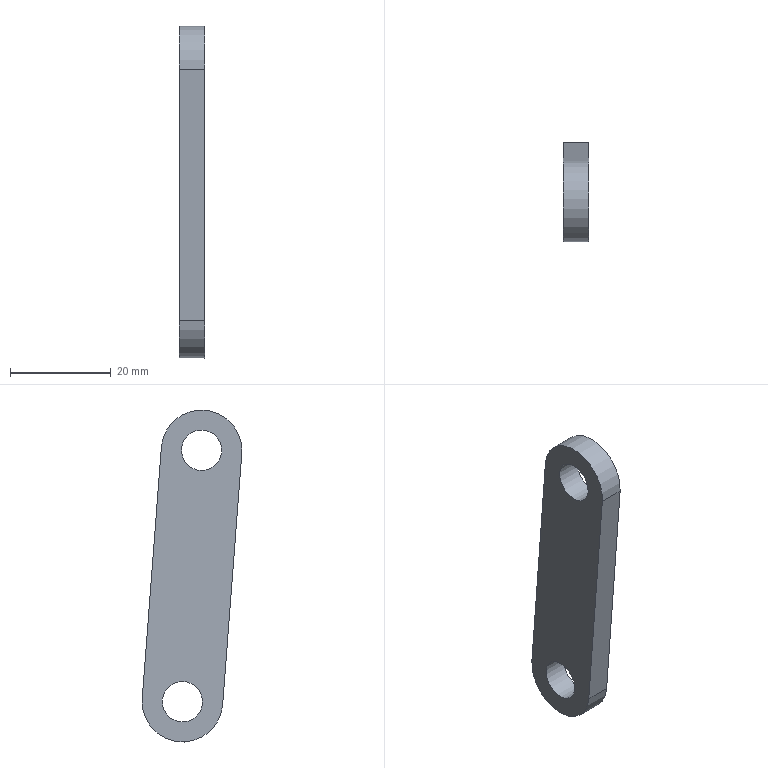Component | NX | JAWLINK2_3 | 1 solid | 8 faces | box 5 x 19.79 x 65.86 mm | volume 4503 mm3 | plane 4 | cylinder 4 | commonest cylinder face diameters 16 x2 8 x2
STEP:
#1=CARTESIAN_POINT('',(0.,0.,0.));
#2=DIRECTION('',(0.,0.,1.));
#3=DIRECTION('',(1.,0.,0.));
#4=AXIS2_PLACEMENT_3D('',#1,#2,#3);
#5=CARTESIAN_POINT('',(-17.89,-45.538,-245.161));
#6=VERTEX_POINT('',#5);
#7=CARTESIAN_POINT('',(-17.89,-41.549,-244.858));
#8=DIRECTION('',(-1.,0.,0.));
#9=DIRECTION('',(0.,-0.9971,-0.07581));
#10=AXIS2_PLACEMENT_3D('',#7,#8,#9);
#11=CIRCLE('',#10,4.);
#12=CARTESIAN_POINT('',(-17.89,-39.654,-269.786));
#13=DIRECTION('',(1.,0.,0.));
#14=DIRECTION('',(0.,0.9971,0.07581));
#15=AXIS2_PLACEMENT_3D('',#12,#13,#14);
#16=PLANE('',#15);
#17=CARTESIAN_POINT('',(-4.,25.));
#18=CARTESIAN_POINT('',(-4.,31.928));
#19=CARTESIAN_POINT('',(2.,28.464));
#20=CARTESIAN_POINT('',(8.,25.));
#21=CARTESIAN_POINT('',(2.,21.536));
#22=CARTESIAN_POINT('',(-4.,18.072));
#23=CARTESIAN_POINT('',(-4.,25.));
#24=(BOUNDED_CURVE()B_SPLINE_CURVE(2,(#17,#18,#19,#20,#21,#22,#23),.UNSPECIFIED.,.T.,.F.)B_SPLINE_CURVE_WITH_KNOTS((1,2,2,2,2,1),(-2.094,0.,2.094,4.189,6.283,8.378),.UNSPECIFIED.)CURVE()GEOMETRIC_REPRESENTATION_ITEM()RATIONAL_B_SPLINE_CURVE((1.,0.5,1.,0.5,1.,0.5,1.))REPRESENTATION_ITEM(''));
#25=(GEOMETRIC_REPRESENTATION_CONTEXT(2)PARAMETRIC_REPRESENTATION_CONTEXT()REPRESENTATION_CONTEXT('',''));
#26=DEFINITIONAL_REPRESENTATION('',(#24),#25);
#27=PCURVE('',#16,#26);
#28=CARTESIAN_POINT('',(-17.89,-41.549,-244.858));
#29=DIRECTION('',(-1.,0.,0.));
#30=DIRECTION('',(0.,-0.9971,-0.07581));
#31=AXIS2_PLACEMENT_3D('',#28,#29,#30);
#32=CYLINDRICAL_SURFACE('',#31,4.);
#33=CARTESIAN_POINT('',(0.,0.));
#34=DIRECTION('',(1.,0.));
#35=VECTOR('',#34,1.);
#36=LINE('',#33,#35);
#37=(GEOMETRIC_REPRESENTATION_CONTEXT(2)PARAMETRIC_REPRESENTATION_CONTEXT()REPRESENTATION_CONTEXT('',''));
#38=DEFINITIONAL_REPRESENTATION('',(#36),#37);
#39=PCURVE('',#32,#38);
#40=SURFACE_CURVE('',#11,(#27,#39),.PCURVE_S1.);
#41=EDGE_CURVE('',#6,#6,#40,.T.);
#42=ORIENTED_EDGE('',*,*,#41,.T.);
#43=EDGE_LOOP('',(#42));
#44=FACE_BOUND('',#43,.T.);
#45=CARTESIAN_POINT('',(-17.89,-41.747,-295.017));
#46=VERTEX_POINT('',#45);
#47=CARTESIAN_POINT('',(-17.89,-37.759,-294.714));
#48=DIRECTION('',(-1.,0.,0.));
#49=DIRECTION('',(0.,-0.9971,-0.07581));
#50=AXIS2_PLACEMENT_3D('',#47,#48,#49);
#51=CIRCLE('',#50,4.);
#52=CARTESIAN_POINT('',(-4.,-25.));
#53=CARTESIAN_POINT('',(-4.,-18.072));
#54=CARTESIAN_POINT('',(2.,-21.536));
#55=CARTESIAN_POINT('',(8.,-25.));
#56=CARTESIAN_POINT('',(2.,-28.464));
#57=CARTESIAN_POINT('',(-4.,-31.928));
#58=CARTESIAN_POINT('',(-4.,-25.));
#59=(BOUNDED_CURVE()B_SPLINE_CURVE(2,(#52,#53,#54,#55,#56,#57,#58),.UNSPECIFIED.,.T.,.F.)B_SPLINE_CURVE_WITH_KNOTS((1,2,2,2,2,1),(-2.094,0.,2.094,4.189,6.283,8.378),.UNSPECIFIED.)CURVE()GEOMETRIC_REPRESENTATION_ITEM()RATIONAL_B_SPLINE_CURVE((1.,0.5,1.,0.5,1.,0.5,1.))REPRESENTATION_ITEM(''));
#60=(GEOMETRIC_REPRESENTATION_CONTEXT(2)PARAMETRIC_REPRESENTATION_CONTEXT()REPRESENTATION_CONTEXT('',''));
#61=DEFINITIONAL_REPRESENTATION('',(#59),#60);
#62=PCURVE('',#16,#61);
#63=CARTESIAN_POINT('',(-17.89,-37.759,-294.714));
#64=DIRECTION('',(-1.,0.,0.));
#65=DIRECTION('',(0.,-0.9971,-0.07581));
#66=AXIS2_PLACEMENT_3D('',#63,#64,#65);
#67=CYLINDRICAL_SURFACE('',#66,4.);
#68=CARTESIAN_POINT('',(0.,0.));
#69=DIRECTION('',(1.,0.));
#70=VECTOR('',#69,1.);
#71=LINE('',#68,#70);
#72=(GEOMETRIC_REPRESENTATION_CONTEXT(2)PARAMETRIC_REPRESENTATION_CONTEXT()REPRESENTATION_CONTEXT('',''));
#73=DEFINITIONAL_REPRESENTATION('',(#71),#72);
#74=PCURVE('',#67,#73);
#75=SURFACE_CURVE('',#51,(#62,#74),.PCURVE_S1.);
#76=EDGE_CURVE('',#46,#46,#75,.T.);
#77=ORIENTED_EDGE('',*,*,#76,.T.);
#78=EDGE_LOOP('',(#77));
#79=FACE_BOUND('',#78,.T.);
#80=CARTESIAN_POINT('',(-17.89,-33.572,-244.251));
#81=VERTEX_POINT('',#80);
#82=CARTESIAN_POINT('',(-17.89,-49.526,-245.464));
#83=VERTEX_POINT('',#82);
#84=CARTESIAN_POINT('',(-17.89,-41.549,-244.858));
#85=DIRECTION('',(1.,0.,0.));
#86=DIRECTION('',(0.,0.9971,0.07581));
#87=AXIS2_PLACEMENT_3D('',#84,#85,#86);
#88=CIRCLE('',#87,8.);
#89=CARTESIAN_POINT('',(-0.,25.));
#90=DIRECTION('',(1.,0.));
#91=AXIS2_PLACEMENT_2D('',#89,#90);
#92=CIRCLE('',#91,8.);
#93=(GEOMETRIC_REPRESENTATION_CONTEXT(2)PARAMETRIC_REPRESENTATION_CONTEXT()REPRESENTATION_CONTEXT('',''));
#94=DEFINITIONAL_REPRESENTATION('',(#92),#93);
#95=PCURVE('',#16,#94);
#96=CARTESIAN_POINT('',(-22.89,-41.549,-244.858));
#97=DIRECTION('',(1.,0.,0.));
#98=DIRECTION('',(0.,0.9971,0.07581));
#99=AXIS2_PLACEMENT_3D('',#96,#97,#98);
#100=CYLINDRICAL_SURFACE('',#99,8.);
#101=CARTESIAN_POINT('',(0.,5.));
#102=DIRECTION('',(1.,0.));
#103=VECTOR('',#102,1.);
#104=LINE('',#101,#103);
#105=(GEOMETRIC_REPRESENTATION_CONTEXT(2)PARAMETRIC_REPRESENTATION_CONTEXT()REPRESENTATION_CONTEXT('',''));
#106=DEFINITIONAL_REPRESENTATION('',(#104),#105);
#107=PCURVE('',#100,#106);
#108=SURFACE_CURVE('',#88,(#95,#107),.PCURVE_S1.);
#109=EDGE_CURVE('',#81,#83,#108,.T.);
#110=ORIENTED_EDGE('',*,*,#109,.T.);
#111=CARTESIAN_POINT('',(-17.89,-45.736,-295.321));
#112=VERTEX_POINT('',#111);
#113=CARTESIAN_POINT('',(-17.89,-47.631,-270.392));
#114=DIRECTION('',(0.,-0.07581,0.9971));
#115=VECTOR('',#114,1.);
#116=LINE('',#113,#115);
#117=CARTESIAN_POINT('',(-8.,-0.));
#118=DIRECTION('',(0.,1.));
#119=VECTOR('',#118,1.);
#120=LINE('',#117,#119);
#121=(GEOMETRIC_REPRESENTATION_CONTEXT(2)PARAMETRIC_REPRESENTATION_CONTEXT()REPRESENTATION_CONTEXT('',''));
#122=DEFINITIONAL_REPRESENTATION('',(#120),#121);
#123=PCURVE('',#16,#122);
#124=CARTESIAN_POINT('',(-22.89,-47.631,-270.392));
#125=DIRECTION('',(0.,-0.9971,-0.07581));
#126=DIRECTION('',(1.,0.,0.));
#127=AXIS2_PLACEMENT_3D('',#124,#125,#126);
#128=PLANE('',#127);
#129=CARTESIAN_POINT('',(5.,0.));
#130=DIRECTION('',(0.,1.));
#131=VECTOR('',#130,1.);
#132=LINE('',#129,#131);
#133=(GEOMETRIC_REPRESENTATION_CONTEXT(2)PARAMETRIC_REPRESENTATION_CONTEXT()REPRESENTATION_CONTEXT('',''));
#134=DEFINITIONAL_REPRESENTATION('',(#132),#133);
#135=PCURVE('',#128,#134);
#136=SURFACE_CURVE('',#116,(#123,#135),.PCURVE_S1.);
#137=EDGE_CURVE('',#112,#83,#136,.T.);
#138=ORIENTED_EDGE('',*,*,#137,.F.);
#139=CARTESIAN_POINT('',(-17.89,-29.782,-294.108));
#140=VERTEX_POINT('',#139);
#141=CARTESIAN_POINT('',(-17.89,-37.759,-294.714));
#142=DIRECTION('',(1.,0.,0.));
#143=DIRECTION('',(0.,0.9971,0.07581));
#144=AXIS2_PLACEMENT_3D('',#141,#142,#143);
#145=CIRCLE('',#144,8.);
#146=CARTESIAN_POINT('',(-0.,-25.));
#147=DIRECTION('',(1.,-0.));
#148=AXIS2_PLACEMENT_2D('',#146,#147);
#149=CIRCLE('',#148,8.);
#150=(GEOMETRIC_REPRESENTATION_CONTEXT(2)PARAMETRIC_REPRESENTATION_CONTEXT()REPRESENTATION_CONTEXT('',''));
#151=DEFINITIONAL_REPRESENTATION('',(#149),#150);
#152=PCURVE('',#16,#151);
#153=CARTESIAN_POINT('',(-22.89,-37.759,-294.714));
#154=DIRECTION('',(1.,0.,0.));
#155=DIRECTION('',(0.,0.9971,0.07581));
#156=AXIS2_PLACEMENT_3D('',#153,#154,#155);
#157=CYLINDRICAL_SURFACE('',#156,8.);
#158=CARTESIAN_POINT('',(0.,5.));
#159=DIRECTION('',(1.,0.));
#160=VECTOR('',#159,1.);
#161=LINE('',#158,#160);
#162=(GEOMETRIC_REPRESENTATION_CONTEXT(2)PARAMETRIC_REPRESENTATION_CONTEXT()REPRESENTATION_CONTEXT('',''));
#163=DEFINITIONAL_REPRESENTATION('',(#161),#162);
#164=PCURVE('',#157,#163);
#165=SURFACE_CURVE('',#145,(#152,#164),.PCURVE_S1.);
#166=EDGE_CURVE('',#112,#140,#165,.T.);
#167=ORIENTED_EDGE('',*,*,#166,.T.);
#168=CARTESIAN_POINT('',(-17.89,-31.677,-269.179));
#169=DIRECTION('',(0.,0.07581,-0.9971));
#170=VECTOR('',#169,1.);
#171=LINE('',#168,#170);
#172=CARTESIAN_POINT('',(8.,0.));
#173=DIRECTION('',(0.,-1.));
#174=VECTOR('',#173,1.);
#175=LINE('',#172,#174);
#176=(GEOMETRIC_REPRESENTATION_CONTEXT(2)PARAMETRIC_REPRESENTATION_CONTEXT()REPRESENTATION_CONTEXT('',''));
#177=DEFINITIONAL_REPRESENTATION('',(#175),#176);
#178=PCURVE('',#16,#177);
#179=CARTESIAN_POINT('',(-22.89,-31.677,-269.179));
#180=DIRECTION('',(0.,0.9971,0.07581));
#181=DIRECTION('',(-1.,0.,0.));
#182=AXIS2_PLACEMENT_3D('',#179,#180,#181);
#183=PLANE('',#182);
#184=CARTESIAN_POINT('',(-5.,0.));
#185=DIRECTION('',(0.,-1.));
#186=VECTOR('',#185,1.);
#187=LINE('',#184,#186);
#188=(GEOMETRIC_REPRESENTATION_CONTEXT(2)PARAMETRIC_REPRESENTATION_CONTEXT()REPRESENTATION_CONTEXT('',''));
#189=DEFINITIONAL_REPRESENTATION('',(#187),#188);
#190=PCURVE('',#183,#189);
#191=SURFACE_CURVE('',#171,(#178,#190),.PCURVE_S1.);
#192=EDGE_CURVE('',#81,#140,#191,.T.);
#193=ORIENTED_EDGE('',*,*,#192,.F.);
#194=EDGE_LOOP('',(#110,#138,#167,#193));
#195=FACE_BOUND('',#194,.T.);
#196=ADVANCED_FACE('',(#44,#79,#195),#16,.T.);
#197=ORIENTED_EDGE('',*,*,#137,.T.);
#198=CARTESIAN_POINT('',(-22.89,-49.526,-245.464));
#199=VERTEX_POINT('',#198);
#200=CARTESIAN_POINT('',(-22.89,-49.526,-245.464));
#201=DIRECTION('',(-1.,0.,0.));
#202=VECTOR('',#201,1.);
#203=LINE('',#200,#202);
#204=CARTESIAN_POINT('',(0.,25.));
#205=DIRECTION('',(-1.,0.));
#206=VECTOR('',#205,1.);
#207=LINE('',#204,#206);
#208=(GEOMETRIC_REPRESENTATION_CONTEXT(2)PARAMETRIC_REPRESENTATION_CONTEXT()REPRESENTATION_CONTEXT('',''));
#209=DEFINITIONAL_REPRESENTATION('',(#207),#208);
#210=PCURVE('',#128,#209);
#211=CARTESIAN_POINT('',(3.142,0.));
#212=DIRECTION('',(0.,-1.));
#213=VECTOR('',#212,1.);
#214=LINE('',#211,#213);
#215=(GEOMETRIC_REPRESENTATION_CONTEXT(2)PARAMETRIC_REPRESENTATION_CONTEXT()REPRESENTATION_CONTEXT('',''));
#216=DEFINITIONAL_REPRESENTATION('',(#214),#215);
#217=PCURVE('',#100,#216);
#218=SURFACE_CURVE('',#203,(#210,#217),.PCURVE_S1.);
#219=EDGE_CURVE('',#83,#199,#218,.T.);
#220=ORIENTED_EDGE('',*,*,#219,.T.);
#221=CARTESIAN_POINT('',(-22.89,-45.736,-295.321));
#222=VERTEX_POINT('',#221);
#223=CARTESIAN_POINT('',(-22.89,-47.631,-270.392));
#224=DIRECTION('',(0.,0.07581,-0.9971));
#225=VECTOR('',#224,1.);
#226=LINE('',#223,#225);
#227=CARTESIAN_POINT('',(0.,0.));
#228=DIRECTION('',(0.,-1.));
#229=VECTOR('',#228,1.);
#230=LINE('',#227,#229);
#231=(GEOMETRIC_REPRESENTATION_CONTEXT(2)PARAMETRIC_REPRESENTATION_CONTEXT()REPRESENTATION_CONTEXT('',''));
#232=DEFINITIONAL_REPRESENTATION('',(#230),#231);
#233=PCURVE('',#128,#232);
#234=CARTESIAN_POINT('',(-22.89,-39.654,-269.786));
#235=DIRECTION('',(-1.,0.,0.));
#236=DIRECTION('',(0.,-0.9971,-0.07581));
#237=AXIS2_PLACEMENT_3D('',#234,#235,#236);
#238=PLANE('',#237);
#239=CARTESIAN_POINT('',(8.,-0.));
#240=DIRECTION('',(0.,-1.));
#241=VECTOR('',#240,1.);
#242=LINE('',#239,#241);
#243=(GEOMETRIC_REPRESENTATION_CONTEXT(2)PARAMETRIC_REPRESENTATION_CONTEXT()REPRESENTATION_CONTEXT('',''));
#244=DEFINITIONAL_REPRESENTATION('',(#242),#243);
#245=PCURVE('',#238,#244);
#246=SURFACE_CURVE('',#226,(#233,#245),.PCURVE_S1.);
#247=EDGE_CURVE('',#199,#222,#246,.T.);
#248=ORIENTED_EDGE('',*,*,#247,.T.);
#249=CARTESIAN_POINT('',(-22.89,-45.736,-295.321));
#250=DIRECTION('',(1.,0.,0.));
#251=VECTOR('',#250,1.);
#252=LINE('',#249,#251);
#253=CARTESIAN_POINT('',(0.,-25.));
#254=DIRECTION('',(1.,0.));
#255=VECTOR('',#254,1.);
#256=LINE('',#253,#255);
#257=(GEOMETRIC_REPRESENTATION_CONTEXT(2)PARAMETRIC_REPRESENTATION_CONTEXT()REPRESENTATION_CONTEXT('',''));
#258=DEFINITIONAL_REPRESENTATION('',(#256),#257);
#259=PCURVE('',#128,#258);
#260=CARTESIAN_POINT('',(3.142,0.));
#261=DIRECTION('',(0.,1.));
#262=VECTOR('',#261,1.);
#263=LINE('',#260,#262);
#264=(GEOMETRIC_REPRESENTATION_CONTEXT(2)PARAMETRIC_REPRESENTATION_CONTEXT()REPRESENTATION_CONTEXT('',''));
#265=DEFINITIONAL_REPRESENTATION('',(#263),#264);
#266=PCURVE('',#157,#265);
#267=SURFACE_CURVE('',#252,(#259,#266),.PCURVE_S1.);
#268=EDGE_CURVE('',#222,#112,#267,.T.);
#269=ORIENTED_EDGE('',*,*,#268,.T.);
#270=EDGE_LOOP('',(#197,#220,#248,#269));
#271=FACE_BOUND('',#270,.T.);
#272=ADVANCED_FACE('',(#271),#128,.T.);
#273=CARTESIAN_POINT('',(-22.89,-45.538,-245.161));
#274=VERTEX_POINT('',#273);
#275=CARTESIAN_POINT('',(-22.89,-41.549,-244.858));
#276=DIRECTION('',(-1.,0.,0.));
#277=DIRECTION('',(0.,-0.9971,-0.07581));
#278=AXIS2_PLACEMENT_3D('',#275,#276,#277);
#279=CIRCLE('',#278,4.);
#280=CARTESIAN_POINT('',(0.,25.));
#281=DIRECTION('',(1.,0.));
#282=AXIS2_PLACEMENT_2D('',#280,#281);
#283=CIRCLE('',#282,4.);
#284=(GEOMETRIC_REPRESENTATION_CONTEXT(2)PARAMETRIC_REPRESENTATION_CONTEXT()REPRESENTATION_CONTEXT('',''));
#285=DEFINITIONAL_REPRESENTATION('',(#283),#284);
#286=PCURVE('',#238,#285);
#287=CARTESIAN_POINT('',(0.,5.));
#288=DIRECTION('',(1.,0.));
#289=VECTOR('',#288,1.);
#290=LINE('',#287,#289);
#291=(GEOMETRIC_REPRESENTATION_CONTEXT(2)PARAMETRIC_REPRESENTATION_CONTEXT()REPRESENTATION_CONTEXT('',''));
#292=DEFINITIONAL_REPRESENTATION('',(#290),#291);
#293=PCURVE('',#32,#292);
#294=SURFACE_CURVE('',#279,(#286,#293),.PCURVE_S1.);
#295=EDGE_CURVE('',#274,#274,#294,.T.);
#296=ORIENTED_EDGE('',*,*,#295,.F.);
#297=EDGE_LOOP('',(#296));
#298=FACE_BOUND('',#297,.T.);
#299=CARTESIAN_POINT('',(-22.89,-41.747,-295.017));
#300=VERTEX_POINT('',#299);
#301=CARTESIAN_POINT('',(-22.89,-37.759,-294.714));
#302=DIRECTION('',(-1.,0.,0.));
#303=DIRECTION('',(0.,-0.9971,-0.07581));
#304=AXIS2_PLACEMENT_3D('',#301,#302,#303);
#305=CIRCLE('',#304,4.);
#306=CARTESIAN_POINT('',(0.,-25.));
#307=DIRECTION('',(1.,-0.));
#308=AXIS2_PLACEMENT_2D('',#306,#307);
#309=CIRCLE('',#308,4.);
#310=(GEOMETRIC_REPRESENTATION_CONTEXT(2)PARAMETRIC_REPRESENTATION_CONTEXT()REPRESENTATION_CONTEXT('',''));
#311=DEFINITIONAL_REPRESENTATION('',(#309),#310);
#312=PCURVE('',#238,#311);
#313=CARTESIAN_POINT('',(0.,5.));
#314=DIRECTION('',(1.,0.));
#315=VECTOR('',#314,1.);
#316=LINE('',#313,#315);
#317=(GEOMETRIC_REPRESENTATION_CONTEXT(2)PARAMETRIC_REPRESENTATION_CONTEXT()REPRESENTATION_CONTEXT('',''));
#318=DEFINITIONAL_REPRESENTATION('',(#316),#317);
#319=PCURVE('',#67,#318);
#320=SURFACE_CURVE('',#305,(#312,#319),.PCURVE_S1.);
#321=EDGE_CURVE('',#300,#300,#320,.T.);
#322=ORIENTED_EDGE('',*,*,#321,.F.);
#323=EDGE_LOOP('',(#322));
#324=FACE_BOUND('',#323,.T.);
#325=ORIENTED_EDGE('',*,*,#247,.F.);
#326=CARTESIAN_POINT('',(-22.89,-33.572,-244.251));
#327=VERTEX_POINT('',#326);
#328=CARTESIAN_POINT('',(-22.89,-41.549,-244.858));
#329=DIRECTION('',(-1.,0.,0.));
#330=DIRECTION('',(0.,-0.9971,-0.07581));
#331=AXIS2_PLACEMENT_3D('',#328,#329,#330);
#332=CIRCLE('',#331,8.);
#333=CARTESIAN_POINT('',(0.,25.));
#334=DIRECTION('',(1.,-0.));
#335=AXIS2_PLACEMENT_2D('',#333,#334);
#336=CIRCLE('',#335,8.);
#337=(GEOMETRIC_REPRESENTATION_CONTEXT(2)PARAMETRIC_REPRESENTATION_CONTEXT()REPRESENTATION_CONTEXT('',''));
#338=DEFINITIONAL_REPRESENTATION('',(#336),#337);
#339=PCURVE('',#238,#338);
#340=CARTESIAN_POINT('',(3.142,0.));
#341=DIRECTION('',(-1.,0.));
#342=VECTOR('',#341,1.);
#343=LINE('',#340,#342);
#344=(GEOMETRIC_REPRESENTATION_CONTEXT(2)PARAMETRIC_REPRESENTATION_CONTEXT()REPRESENTATION_CONTEXT('',''));
#345=DEFINITIONAL_REPRESENTATION('',(#343),#344);
#346=PCURVE('',#100,#345);
#347=SURFACE_CURVE('',#332,(#339,#346),.PCURVE_S1.);
#348=EDGE_CURVE('',#199,#327,#347,.T.);
#349=ORIENTED_EDGE('',*,*,#348,.T.);
#350=CARTESIAN_POINT('',(-22.89,-29.782,-294.108));
#351=VERTEX_POINT('',#350);
#352=CARTESIAN_POINT('',(-22.89,-31.677,-269.179));
#353=DIRECTION('',(0.,-0.07581,0.9971));
#354=VECTOR('',#353,1.);
#355=LINE('',#352,#354);
#356=CARTESIAN_POINT('',(-8.,0.));
#357=DIRECTION('',(0.,1.));
#358=VECTOR('',#357,1.);
#359=LINE('',#356,#358);
#360=(GEOMETRIC_REPRESENTATION_CONTEXT(2)PARAMETRIC_REPRESENTATION_CONTEXT()REPRESENTATION_CONTEXT('',''));
#361=DEFINITIONAL_REPRESENTATION('',(#359),#360);
#362=PCURVE('',#238,#361);
#363=CARTESIAN_POINT('',(0.,0.));
#364=DIRECTION('',(0.,1.));
#365=VECTOR('',#364,1.);
#366=LINE('',#363,#365);
#367=(GEOMETRIC_REPRESENTATION_CONTEXT(2)PARAMETRIC_REPRESENTATION_CONTEXT()REPRESENTATION_CONTEXT('',''));
#368=DEFINITIONAL_REPRESENTATION('',(#366),#367);
#369=PCURVE('',#183,#368);
#370=SURFACE_CURVE('',#355,(#362,#369),.PCURVE_S1.);
#371=EDGE_CURVE('',#351,#327,#370,.T.);
#372=ORIENTED_EDGE('',*,*,#371,.F.);
#373=CARTESIAN_POINT('',(-22.89,-37.759,-294.714));
#374=DIRECTION('',(-1.,0.,0.));
#375=DIRECTION('',(0.,-0.9971,-0.07581));
#376=AXIS2_PLACEMENT_3D('',#373,#374,#375);
#377=CIRCLE('',#376,8.);
#378=CARTESIAN_POINT('',(0.,-25.));
#379=DIRECTION('',(1.,0.));
#380=AXIS2_PLACEMENT_2D('',#378,#379);
#381=CIRCLE('',#380,8.);
#382=(GEOMETRIC_REPRESENTATION_CONTEXT(2)PARAMETRIC_REPRESENTATION_CONTEXT()REPRESENTATION_CONTEXT('',''));
#383=DEFINITIONAL_REPRESENTATION('',(#381),#382);
#384=PCURVE('',#238,#383);
#385=CARTESIAN_POINT('',(9.425,0.));
#386=DIRECTION('',(-1.,0.));
#387=VECTOR('',#386,1.);
#388=LINE('',#385,#387);
#389=(GEOMETRIC_REPRESENTATION_CONTEXT(2)PARAMETRIC_REPRESENTATION_CONTEXT()REPRESENTATION_CONTEXT('',''));
#390=DEFINITIONAL_REPRESENTATION('',(#388),#389);
#391=PCURVE('',#157,#390);
#392=SURFACE_CURVE('',#377,(#384,#391),.PCURVE_S1.);
#393=EDGE_CURVE('',#351,#222,#392,.T.);
#394=ORIENTED_EDGE('',*,*,#393,.T.);
#395=EDGE_LOOP('',(#325,#349,#372,#394));
#396=FACE_BOUND('',#395,.T.);
#397=ADVANCED_FACE('',(#298,#324,#396),#238,.T.);
#398=ORIENTED_EDGE('',*,*,#371,.T.);
#399=CARTESIAN_POINT('',(-22.89,-33.572,-244.251));
#400=DIRECTION('',(1.,0.,0.));
#401=VECTOR('',#400,1.);
#402=LINE('',#399,#401);
#403=CARTESIAN_POINT('',(0.,25.));
#404=DIRECTION('',(-1.,0.));
#405=VECTOR('',#404,1.);
#406=LINE('',#403,#405);
#407=(GEOMETRIC_REPRESENTATION_CONTEXT(2)PARAMETRIC_REPRESENTATION_CONTEXT()REPRESENTATION_CONTEXT('',''));
#408=DEFINITIONAL_REPRESENTATION('',(#406),#407);
#409=PCURVE('',#183,#408);
#410=CARTESIAN_POINT('',(0.,0.));
#411=DIRECTION('',(0.,1.));
#412=VECTOR('',#411,1.);
#413=LINE('',#410,#412);
#414=(GEOMETRIC_REPRESENTATION_CONTEXT(2)PARAMETRIC_REPRESENTATION_CONTEXT()REPRESENTATION_CONTEXT('',''));
#415=DEFINITIONAL_REPRESENTATION('',(#413),#414);
#416=PCURVE('',#100,#415);
#417=SURFACE_CURVE('',#402,(#409,#416),.PCURVE_S1.);
#418=EDGE_CURVE('',#327,#81,#417,.T.);
#419=ORIENTED_EDGE('',*,*,#418,.T.);
#420=ORIENTED_EDGE('',*,*,#192,.T.);
#421=CARTESIAN_POINT('',(-22.89,-29.782,-294.108));
#422=DIRECTION('',(-1.,0.,0.));
#423=VECTOR('',#422,1.);
#424=LINE('',#421,#423);
#425=CARTESIAN_POINT('',(0.,-25.));
#426=DIRECTION('',(1.,0.));
#427=VECTOR('',#426,1.);
#428=LINE('',#425,#427);
#429=(GEOMETRIC_REPRESENTATION_CONTEXT(2)PARAMETRIC_REPRESENTATION_CONTEXT()REPRESENTATION_CONTEXT('',''));
#430=DEFINITIONAL_REPRESENTATION('',(#428),#429);
#431=PCURVE('',#183,#430);
#432=CARTESIAN_POINT('',(6.283,0.));
#433=DIRECTION('',(0.,-1.));
#434=VECTOR('',#433,1.);
#435=LINE('',#432,#434);
#436=(GEOMETRIC_REPRESENTATION_CONTEXT(2)PARAMETRIC_REPRESENTATION_CONTEXT()REPRESENTATION_CONTEXT('',''));
#437=DEFINITIONAL_REPRESENTATION('',(#435),#436);
#438=PCURVE('',#157,#437);
#439=SURFACE_CURVE('',#424,(#431,#438),.PCURVE_S1.);
#440=EDGE_CURVE('',#140,#351,#439,.T.);
#441=ORIENTED_EDGE('',*,*,#440,.T.);
#442=EDGE_LOOP('',(#398,#419,#420,#441));
#443=FACE_BOUND('',#442,.T.);
#444=ADVANCED_FACE('',(#443),#183,.T.);
#445=ORIENTED_EDGE('',*,*,#418,.F.);
#446=ORIENTED_EDGE('',*,*,#348,.F.);
#447=ORIENTED_EDGE('',*,*,#219,.F.);
#448=ORIENTED_EDGE('',*,*,#109,.F.);
#449=EDGE_LOOP('',(#445,#446,#447,#448));
#450=FACE_BOUND('',#449,.T.);
#451=ADVANCED_FACE('',(#450),#100,.T.);
#452=ORIENTED_EDGE('',*,*,#166,.F.);
#453=ORIENTED_EDGE('',*,*,#268,.F.);
#454=ORIENTED_EDGE('',*,*,#393,.F.);
#455=ORIENTED_EDGE('',*,*,#440,.F.);
#456=EDGE_LOOP('',(#452,#453,#454,#455));
#457=FACE_BOUND('',#456,.T.);
#458=ADVANCED_FACE('',(#457),#157,.T.);
#459=ORIENTED_EDGE('',*,*,#321,.F.);
#460=CARTESIAN_POINT('',(-17.89,-41.747,-295.017));
#461=CARTESIAN_POINT('',(-22.89,-41.747,-295.017));
#462=B_SPLINE_CURVE_WITH_KNOTS('',1,(#460,#461),.UNSPECIFIED.,.F.,.F.,(2,2),(0.,5.),.PIECEWISE_BEZIER_KNOTS.);
#463=CARTESIAN_POINT('',(0.,0.));
#464=DIRECTION('',(0.,1.));
#465=VECTOR('',#464,1.);
#466=LINE('',#463,#465);
#467=(GEOMETRIC_REPRESENTATION_CONTEXT(2)PARAMETRIC_REPRESENTATION_CONTEXT()REPRESENTATION_CONTEXT('',''));
#468=DEFINITIONAL_REPRESENTATION('',(#466),#467);
#469=PCURVE('',#67,#468);
#470=CARTESIAN_POINT('',(6.283,0.));
#471=DIRECTION('',(0.,1.));
#472=VECTOR('',#471,1.);
#473=LINE('',#470,#472);
#474=(GEOMETRIC_REPRESENTATION_CONTEXT(2)PARAMETRIC_REPRESENTATION_CONTEXT()REPRESENTATION_CONTEXT('',''));
#475=DEFINITIONAL_REPRESENTATION('',(#473),#474);
#476=PCURVE('',#67,#475);
#477=SEAM_CURVE('',#462,(#469,#476),.PCURVE_S1.);
#478=EDGE_CURVE('',#46,#300,#477,.T.);
#479=ORIENTED_EDGE('',*,*,#478,.F.);
#480=ORIENTED_EDGE('',*,*,#76,.T.);
#481=ORIENTED_EDGE('',*,*,#478,.T.);
#482=EDGE_LOOP('',(#459,#479,#480,#481));
#483=FACE_BOUND('',#482,.F.);
#484=ADVANCED_FACE('',(#483),#67,.F.);
#485=ORIENTED_EDGE('',*,*,#295,.F.);
#486=CARTESIAN_POINT('',(-17.89,-45.538,-245.161));
#487=CARTESIAN_POINT('',(-22.89,-45.538,-245.161));
#488=B_SPLINE_CURVE_WITH_KNOTS('',1,(#486,#487),.UNSPECIFIED.,.F.,.F.,(2,2),(0.,5.),.PIECEWISE_BEZIER_KNOTS.);
#489=CARTESIAN_POINT('',(0.,0.));
#490=DIRECTION('',(0.,1.));
#491=VECTOR('',#490,1.);
#492=LINE('',#489,#491);
#493=(GEOMETRIC_REPRESENTATION_CONTEXT(2)PARAMETRIC_REPRESENTATION_CONTEXT()REPRESENTATION_CONTEXT('',''));
#494=DEFINITIONAL_REPRESENTATION('',(#492),#493);
#495=PCURVE('',#32,#494);
#496=CARTESIAN_POINT('',(6.283,0.));
#497=DIRECTION('',(0.,1.));
#498=VECTOR('',#497,1.);
#499=LINE('',#496,#498);
#500=(GEOMETRIC_REPRESENTATION_CONTEXT(2)PARAMETRIC_REPRESENTATION_CONTEXT()REPRESENTATION_CONTEXT('',''));
#501=DEFINITIONAL_REPRESENTATION('',(#499),#500);
#502=PCURVE('',#32,#501);
#503=SEAM_CURVE('',#488,(#495,#502),.PCURVE_S1.);
#504=EDGE_CURVE('',#6,#274,#503,.T.);
#505=ORIENTED_EDGE('',*,*,#504,.F.);
#506=ORIENTED_EDGE('',*,*,#41,.T.);
#507=ORIENTED_EDGE('',*,*,#504,.T.);
#508=EDGE_LOOP('',(#485,#505,#506,#507));
#509=FACE_BOUND('',#508,.F.);
#510=ADVANCED_FACE('',(#509),#32,.F.);
#511=CLOSED_SHELL('',(#196,#272,#397,#444,#451,#458,#484,#510));
#512=MANIFOLD_SOLID_BREP('',#511);
#513=(LENGTH_UNIT()NAMED_UNIT(*)SI_UNIT(.MILLI.,.METRE.));
#514=UNCERTAINTY_MEASURE_WITH_UNIT(LENGTH_MEASURE(0.000002),#513,'','');
#515=(NAMED_UNIT(*)PLANE_ANGLE_UNIT()SI_UNIT($,.RADIAN.));
#516=(NAMED_UNIT(*)SI_UNIT($,.STERADIAN.)SOLID_ANGLE_UNIT());
#517=(GEOMETRIC_REPRESENTATION_CONTEXT(3)GLOBAL_UNCERTAINTY_ASSIGNED_CONTEXT((#514))GLOBAL_UNIT_ASSIGNED_CONTEXT((#513,#515,#516))REPRESENTATION_CONTEXT('',''));
#518=ADVANCED_BREP_SHAPE_REPRESENTATION('',(#4,#512),#517);